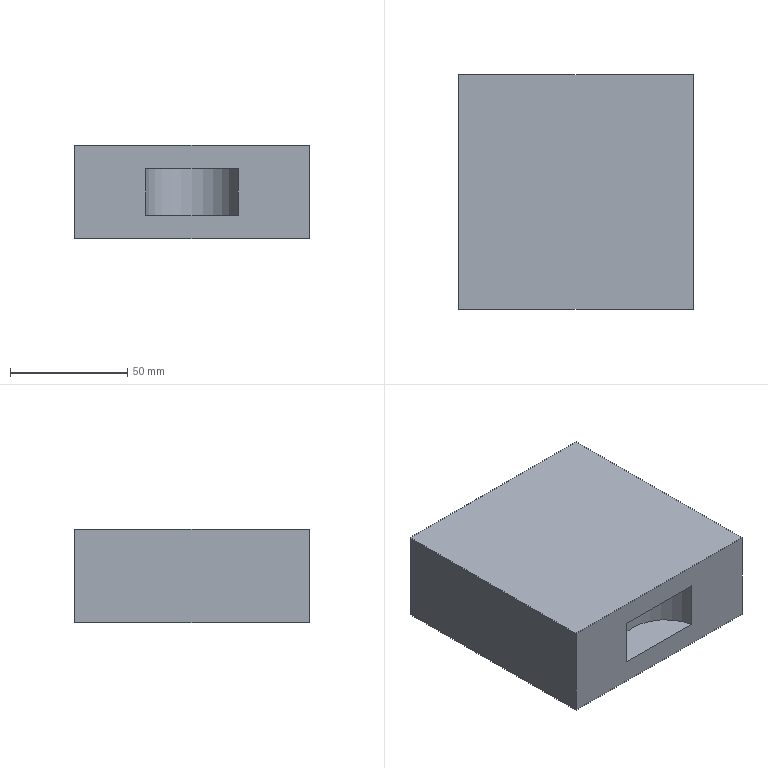CAM job | NX | mm | 3-axis | 1 set-up | 2 operations | part box 100 x 100 x 40
set-up 1
1. Planar Milling | Tcutter Undefined T20 | PLANAR_MILL | path 940.347 mm | 2.693 min
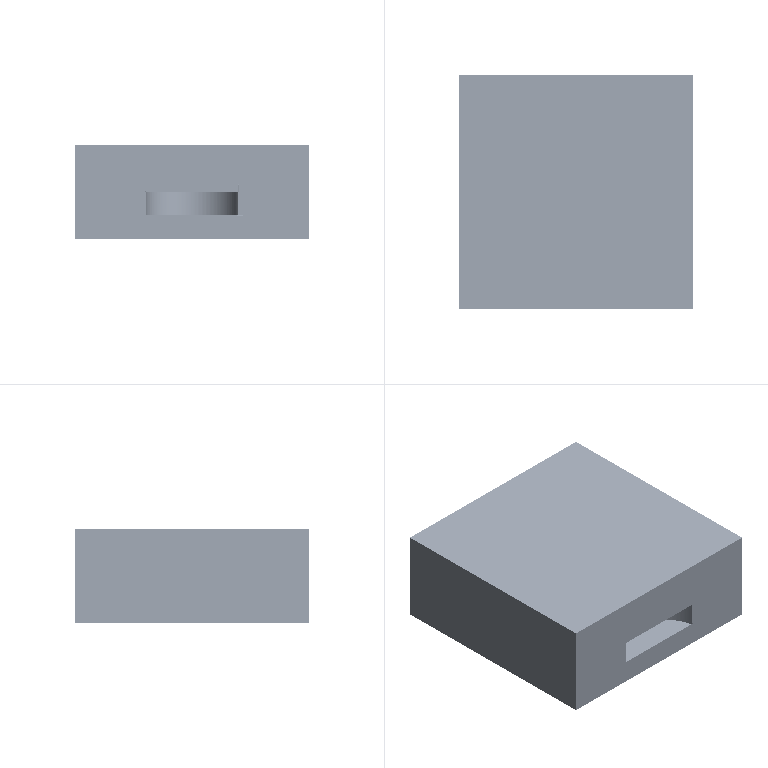2. Planar Milling | Tcutter Undefined T20 | PROFILE_3D | path 226.795 mm | 0.05448 min